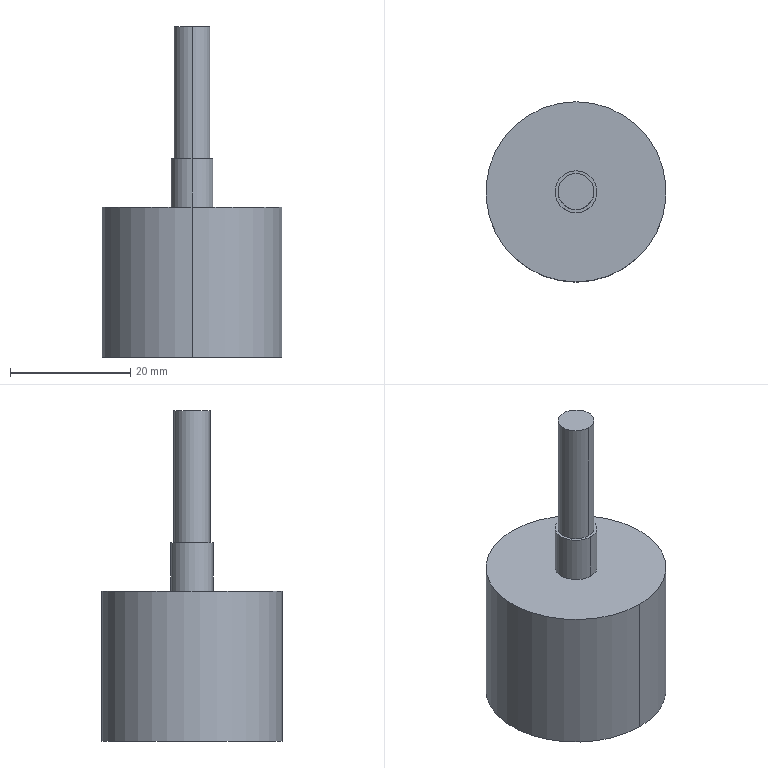Component | SolidWorks | LockingWheel-2 | 1 solid | 10 faces | box 30 x 30 x 55 mm | volume 18601 mm3 | cylinder 6 | plane 4 | commonest cylinder face diameters 6 x2 7 x2 30 x2
build123d program:
from build123d import *


with BuildPart() as part:
    # Sketch1 → Revolve1 (revolve)
    with BuildSketch(Plane.XY, mode=Mode.PRIVATE) as revolve1_sk:
        Polygon((0, 35.261), (15, 35.261), (15, 10.261), (3.5, 10.261), (3.5, 2.261), (3, 2.261), (3, -19.739), (0, -19.739), align=None)
    revolve(revolve1_sk.sketch.rotate(Axis((0, 0, 0), (0, 1, 0)), 90), axis=Axis((0, 0, 0), (0, 1, 0)))


solid = part.part

# Placed as in the assembly
solid = solid.moved(Location((-114.784, 711.983, -103.239), (-90, 0, 0)))
STEP:
#1=CARTESIAN_POINT('',(-4.519,27.913,-4.154));
#2=VERTEX_POINT('',#1);
#3=CARTESIAN_POINT('',(-4.519,28.149,-4.154));
#4=VERTEX_POINT('',#3);
#5=CARTESIAN_POINT('',(-4.519,28.031,-4.154));
#6=DIRECTION('',(0.,0.,1.));
#7=DIRECTION('',(0.,-1.,0.));
#8=AXIS2_PLACEMENT_3D('',#5,#6,#7);
#9=CIRCLE('',#8,0.1181);
#10=EDGE_CURVE('',#2,#4,#9,.T.);
#11=ORIENTED_EDGE('',*,*,#10,.T.);
#12=CARTESIAN_POINT('',(-4.519,28.149,-3.287));
#13=VERTEX_POINT('',#12);
#14=CARTESIAN_POINT('',(-4.519,28.149,-4.065));
#15=DIRECTION('',(0.,0.,1.));
#16=VECTOR('',#15,39.37);
#17=LINE('',#14,#16);
#18=EDGE_CURVE('',#4,#13,#17,.T.);
#19=ORIENTED_EDGE('',*,*,#18,.T.);
#20=CARTESIAN_POINT('',(-4.519,27.913,-3.287));
#21=VERTEX_POINT('',#20);
#22=CARTESIAN_POINT('',(-4.519,28.031,-3.287));
#23=DIRECTION('',(0.,0.,1.));
#24=DIRECTION('',(0.,-1.,0.));
#25=AXIS2_PLACEMENT_3D('',#22,#23,#24);
#26=CIRCLE('',#25,0.1181);
#27=EDGE_CURVE('',#21,#13,#26,.T.);
#28=ORIENTED_EDGE('',*,*,#27,.F.);
#29=CARTESIAN_POINT('',(-4.519,27.913,-4.065));
#30=DIRECTION('',(0.,0.,1.));
#31=VECTOR('',#30,39.37);
#32=LINE('',#29,#31);
#33=EDGE_CURVE('',#2,#21,#32,.T.);
#34=ORIENTED_EDGE('',*,*,#33,.F.);
#35=EDGE_LOOP('',(#11,#19,#28,#34));
#36=FACE_OUTER_BOUND('',#35,.T.);
#37=CARTESIAN_POINT('',(-4.519,28.031,-4.065));
#38=DIRECTION('',(0.,0.,1.));
#39=DIRECTION('',(0.,-1.,0.));
#40=AXIS2_PLACEMENT_3D('',#37,#38,#39);
#41=CYLINDRICAL_SURFACE('',#40,0.1181);
#42=ADVANCED_FACE('',(#36),#41,.T.);
#43=CARTESIAN_POINT('',(-4.519,27.893,-4.469));
#44=VERTEX_POINT('',#43);
#45=CARTESIAN_POINT('',(-4.519,28.169,-4.469));
#46=VERTEX_POINT('',#45);
#47=CARTESIAN_POINT('',(-4.519,28.031,-4.469));
#48=DIRECTION('',(0.,0.,1.));
#49=DIRECTION('',(0.,-1.,0.));
#50=AXIS2_PLACEMENT_3D('',#47,#48,#49);
#51=CIRCLE('',#50,0.1378);
#52=EDGE_CURVE('',#44,#46,#51,.T.);
#53=ORIENTED_EDGE('',*,*,#52,.T.);
#54=CARTESIAN_POINT('',(-4.519,28.169,-4.154));
#55=VERTEX_POINT('',#54);
#56=CARTESIAN_POINT('',(-4.519,28.169,-4.065));
#57=DIRECTION('',(0.,0.,1.));
#58=VECTOR('',#57,39.37);
#59=LINE('',#56,#58);
#60=EDGE_CURVE('',#46,#55,#59,.T.);
#61=ORIENTED_EDGE('',*,*,#60,.T.);
#62=CARTESIAN_POINT('',(-4.519,27.893,-4.154));
#63=VERTEX_POINT('',#62);
#64=CARTESIAN_POINT('',(-4.519,28.031,-4.154));
#65=DIRECTION('',(0.,0.,1.));
#66=DIRECTION('',(0.,-1.,0.));
#67=AXIS2_PLACEMENT_3D('',#64,#65,#66);
#68=CIRCLE('',#67,0.1378);
#69=EDGE_CURVE('',#63,#55,#68,.T.);
#70=ORIENTED_EDGE('',*,*,#69,.F.);
#71=CARTESIAN_POINT('',(-4.519,27.893,-4.065));
#72=DIRECTION('',(0.,0.,1.));
#73=VECTOR('',#72,39.37);
#74=LINE('',#71,#73);
#75=EDGE_CURVE('',#44,#63,#74,.T.);
#76=ORIENTED_EDGE('',*,*,#75,.F.);
#77=EDGE_LOOP('',(#53,#61,#70,#76));
#78=FACE_OUTER_BOUND('',#77,.T.);
#79=CARTESIAN_POINT('',(-4.519,28.031,-4.065));
#80=DIRECTION('',(0.,0.,1.));
#81=DIRECTION('',(0.,-1.,0.));
#82=AXIS2_PLACEMENT_3D('',#79,#80,#81);
#83=CYLINDRICAL_SURFACE('',#82,0.1378);
#84=ADVANCED_FACE('',(#78),#83,.T.);
#85=CARTESIAN_POINT('',(-4.519,27.44,-5.453));
#86=VERTEX_POINT('',#85);
#87=CARTESIAN_POINT('',(-4.519,28.621,-5.453));
#88=VERTEX_POINT('',#87);
#89=CARTESIAN_POINT('',(-4.519,28.031,-5.453));
#90=DIRECTION('',(0.,0.,1.));
#91=DIRECTION('',(0.,-1.,0.));
#92=AXIS2_PLACEMENT_3D('',#89,#90,#91);
#93=CIRCLE('',#92,0.5906);
#94=EDGE_CURVE('',#86,#88,#93,.T.);
#95=ORIENTED_EDGE('',*,*,#94,.T.);
#96=CARTESIAN_POINT('',(-4.519,28.621,-4.469));
#97=VERTEX_POINT('',#96);
#98=CARTESIAN_POINT('',(-4.519,28.621,-4.065));
#99=DIRECTION('',(0.,0.,1.));
#100=VECTOR('',#99,39.37);
#101=LINE('',#98,#100);
#102=EDGE_CURVE('',#88,#97,#101,.T.);
#103=ORIENTED_EDGE('',*,*,#102,.T.);
#104=CARTESIAN_POINT('',(-4.519,27.44,-4.469));
#105=VERTEX_POINT('',#104);
#106=CARTESIAN_POINT('',(-4.519,28.031,-4.469));
#107=DIRECTION('',(0.,0.,1.));
#108=DIRECTION('',(0.,-1.,0.));
#109=AXIS2_PLACEMENT_3D('',#106,#107,#108);
#110=CIRCLE('',#109,0.5906);
#111=EDGE_CURVE('',#105,#97,#110,.T.);
#112=ORIENTED_EDGE('',*,*,#111,.F.);
#113=CARTESIAN_POINT('',(-4.519,27.44,-4.065));
#114=DIRECTION('',(0.,0.,1.));
#115=VECTOR('',#114,39.37);
#116=LINE('',#113,#115);
#117=EDGE_CURVE('',#86,#105,#116,.T.);
#118=ORIENTED_EDGE('',*,*,#117,.F.);
#119=EDGE_LOOP('',(#95,#103,#112,#118));
#120=FACE_OUTER_BOUND('',#119,.T.);
#121=CARTESIAN_POINT('',(-4.519,28.031,-4.065));
#122=DIRECTION('',(0.,0.,1.));
#123=DIRECTION('',(0.,-1.,0.));
#124=AXIS2_PLACEMENT_3D('',#121,#122,#123);
#125=CYLINDRICAL_SURFACE('',#124,0.5906);
#126=ADVANCED_FACE('',(#120),#125,.T.);
#127=ORIENTED_EDGE('',*,*,#94,.F.);
#128=CARTESIAN_POINT('',(-4.519,28.031,-5.453));
#129=DIRECTION('',(0.,0.,1.));
#130=DIRECTION('',(0.,-1.,0.));
#131=AXIS2_PLACEMENT_3D('',#128,#129,#130);
#132=CIRCLE('',#131,0.5906);
#133=EDGE_CURVE('',#88,#86,#132,.T.);
#134=ORIENTED_EDGE('',*,*,#133,.F.);
#135=EDGE_LOOP('',(#127,#134));
#136=FACE_OUTER_BOUND('',#135,.T.);
#137=CARTESIAN_POINT('',(-4.519,28.031,-5.453));
#138=DIRECTION('',(-0.,-0.,-1.));
#139=DIRECTION('',(-0.,1.,-0.));
#140=AXIS2_PLACEMENT_3D('',#137,#138,#139);
#141=PLANE('',#140);
#142=ADVANCED_FACE('',(#136),#141,.T.);
#143=ORIENTED_EDGE('',*,*,#102,.F.);
#144=ORIENTED_EDGE('',*,*,#133,.T.);
#145=ORIENTED_EDGE('',*,*,#117,.T.);
#146=CARTESIAN_POINT('',(-4.519,28.031,-4.469));
#147=DIRECTION('',(0.,0.,1.));
#148=DIRECTION('',(0.,-1.,0.));
#149=AXIS2_PLACEMENT_3D('',#146,#147,#148);
#150=CIRCLE('',#149,0.5906);
#151=EDGE_CURVE('',#97,#105,#150,.T.);
#152=ORIENTED_EDGE('',*,*,#151,.F.);
#153=EDGE_LOOP('',(#143,#144,#145,#152));
#154=FACE_OUTER_BOUND('',#153,.T.);
#155=CARTESIAN_POINT('',(-4.519,28.031,-4.065));
#156=DIRECTION('',(0.,0.,1.));
#157=DIRECTION('',(0.,-1.,0.));
#158=AXIS2_PLACEMENT_3D('',#155,#156,#157);
#159=CYLINDRICAL_SURFACE('',#158,0.5906);
#160=ADVANCED_FACE('',(#154),#159,.T.);
#161=ORIENTED_EDGE('',*,*,#111,.T.);
#162=ORIENTED_EDGE('',*,*,#151,.T.);
#163=EDGE_LOOP('',(#161,#162));
#164=FACE_OUTER_BOUND('',#163,.T.);
#165=ORIENTED_EDGE('',*,*,#52,.F.);
#166=CARTESIAN_POINT('',(-4.519,28.031,-4.469));
#167=DIRECTION('',(0.,0.,1.));
#168=DIRECTION('',(0.,-1.,0.));
#169=AXIS2_PLACEMENT_3D('',#166,#167,#168);
#170=CIRCLE('',#169,0.1378);
#171=EDGE_CURVE('',#46,#44,#170,.T.);
#172=ORIENTED_EDGE('',*,*,#171,.F.);
#173=EDGE_LOOP('',(#165,#172));
#174=FACE_BOUND('',#173,.T.);
#175=CARTESIAN_POINT('',(-3.928,28.031,-4.469));
#176=DIRECTION('',(0.,0.,1.));
#177=DIRECTION('',(0.,-1.,0.));
#178=AXIS2_PLACEMENT_3D('',#175,#176,#177);
#179=PLANE('',#178);
#180=ADVANCED_FACE('',(#164,#174),#179,.T.);
#181=ORIENTED_EDGE('',*,*,#60,.F.);
#182=ORIENTED_EDGE('',*,*,#171,.T.);
#183=ORIENTED_EDGE('',*,*,#75,.T.);
#184=CARTESIAN_POINT('',(-4.519,28.031,-4.154));
#185=DIRECTION('',(0.,0.,1.));
#186=DIRECTION('',(0.,-1.,0.));
#187=AXIS2_PLACEMENT_3D('',#184,#185,#186);
#188=CIRCLE('',#187,0.1378);
#189=EDGE_CURVE('',#55,#63,#188,.T.);
#190=ORIENTED_EDGE('',*,*,#189,.F.);
#191=EDGE_LOOP('',(#181,#182,#183,#190));
#192=FACE_OUTER_BOUND('',#191,.T.);
#193=CARTESIAN_POINT('',(-4.519,28.031,-4.065));
#194=DIRECTION('',(0.,0.,1.));
#195=DIRECTION('',(0.,-1.,0.));
#196=AXIS2_PLACEMENT_3D('',#193,#194,#195);
#197=CYLINDRICAL_SURFACE('',#196,0.1378);
#198=ADVANCED_FACE('',(#192),#197,.T.);
#199=ORIENTED_EDGE('',*,*,#69,.T.);
#200=ORIENTED_EDGE('',*,*,#189,.T.);
#201=EDGE_LOOP('',(#199,#200));
#202=FACE_OUTER_BOUND('',#201,.T.);
#203=ORIENTED_EDGE('',*,*,#10,.F.);
#204=CARTESIAN_POINT('',(-4.519,28.031,-4.154));
#205=DIRECTION('',(0.,0.,1.));
#206=DIRECTION('',(0.,-1.,0.));
#207=AXIS2_PLACEMENT_3D('',#204,#205,#206);
#208=CIRCLE('',#207,0.1181);
#209=EDGE_CURVE('',#4,#2,#208,.T.);
#210=ORIENTED_EDGE('',*,*,#209,.F.);
#211=EDGE_LOOP('',(#203,#210));
#212=FACE_BOUND('',#211,.T.);
#213=CARTESIAN_POINT('',(-4.381,28.031,-4.154));
#214=DIRECTION('',(0.,0.,1.));
#215=DIRECTION('',(0.,-1.,0.));
#216=AXIS2_PLACEMENT_3D('',#213,#214,#215);
#217=PLANE('',#216);
#218=ADVANCED_FACE('',(#202,#212),#217,.T.);
#219=ORIENTED_EDGE('',*,*,#18,.F.);
#220=ORIENTED_EDGE('',*,*,#209,.T.);
#221=ORIENTED_EDGE('',*,*,#33,.T.);
#222=CARTESIAN_POINT('',(-4.519,28.031,-3.287));
#223=DIRECTION('',(0.,0.,1.));
#224=DIRECTION('',(0.,-1.,0.));
#225=AXIS2_PLACEMENT_3D('',#222,#223,#224);
#226=CIRCLE('',#225,0.1181);
#227=EDGE_CURVE('',#13,#21,#226,.T.);
#228=ORIENTED_EDGE('',*,*,#227,.F.);
#229=EDGE_LOOP('',(#219,#220,#221,#228));
#230=FACE_OUTER_BOUND('',#229,.T.);
#231=CARTESIAN_POINT('',(-4.519,28.031,-4.065));
#232=DIRECTION('',(0.,0.,1.));
#233=DIRECTION('',(0.,-1.,0.));
#234=AXIS2_PLACEMENT_3D('',#231,#232,#233);
#235=CYLINDRICAL_SURFACE('',#234,0.1181);
#236=ADVANCED_FACE('',(#230),#235,.T.);
#237=ORIENTED_EDGE('',*,*,#27,.T.);
#238=ORIENTED_EDGE('',*,*,#227,.T.);
#239=EDGE_LOOP('',(#237,#238));
#240=FACE_OUTER_BOUND('',#239,.T.);
#241=CARTESIAN_POINT('',(-4.401,28.031,-3.287));
#242=DIRECTION('',(0.,0.,1.));
#243=DIRECTION('',(0.,-1.,0.));
#244=AXIS2_PLACEMENT_3D('',#241,#242,#243);
#245=PLANE('',#244);
#246=ADVANCED_FACE('',(#240),#245,.T.);
#247=CLOSED_SHELL('',(#42,#84,#126,#142,#160,#180,#198,#218,#236,#246));
#248=MANIFOLD_SOLID_BREP('',#247);
#249=CARTESIAN_POINT('',(0.,0.,0.));
#250=DIRECTION('',(0.,0.,1.));
#251=DIRECTION('',(1.,0.,0.));
#252=AXIS2_PLACEMENT_3D('',#249,#250,#251);
#253=(LENGTH_UNIT()NAMED_UNIT(*)SI_UNIT($,.METRE.));
#254=LENGTH_MEASURE_WITH_UNIT(LENGTH_MEASURE(0.0254),#253);
#255=DIMENSIONAL_EXPONENTS(1.,0.,0.,0.,0.,0.,0.);
#256=(CONVERSION_BASED_UNIT('',#254)LENGTH_UNIT()NAMED_UNIT(#255));
#257=UNCERTAINTY_MEASURE_WITH_UNIT(LENGTH_MEASURE(0.00001),#256,'','');
#258=(NAMED_UNIT(*)PLANE_ANGLE_UNIT()SI_UNIT($,.RADIAN.));
#259=(NAMED_UNIT(*)SI_UNIT($,.STERADIAN.)SOLID_ANGLE_UNIT());
#260=(GEOMETRIC_REPRESENTATION_CONTEXT(3)GLOBAL_UNCERTAINTY_ASSIGNED_CONTEXT((#257))GLOBAL_UNIT_ASSIGNED_CONTEXT((#256,#258,#259))REPRESENTATION_CONTEXT('',''));
#261=ADVANCED_BREP_SHAPE_REPRESENTATION('',(#248,#252),#260);
#262=COLOUR_RGB('',0.7922,0.8196,0.9333);
#263=FILL_AREA_STYLE_COLOUR('',#262);
#264=FILL_AREA_STYLE('',(#263));
#265=SURFACE_STYLE_FILL_AREA(#264);
#266=SURFACE_SIDE_STYLE('',(#265));
#267=SURFACE_STYLE_USAGE(.BOTH.,#266);
#268=PRESENTATION_STYLE_ASSIGNMENT((#267));
#269=STYLED_ITEM('',(#268),#248);
#270=PRESENTATION_LAYER_ASSIGNMENT('','',(#269));
#271=(LENGTH_UNIT()NAMED_UNIT(*)SI_UNIT($,.METRE.));
#272=LENGTH_MEASURE_WITH_UNIT(LENGTH_MEASURE(0.0254),#271);
#273=DIMENSIONAL_EXPONENTS(1.,0.,0.,0.,0.,0.,0.);
#274=(CONVERSION_BASED_UNIT('',#272)LENGTH_UNIT()NAMED_UNIT(#273));
#275=UNCERTAINTY_MEASURE_WITH_UNIT(LENGTH_MEASURE(0.00001),#274,'','');
#276=(NAMED_UNIT(*)PLANE_ANGLE_UNIT()SI_UNIT($,.RADIAN.));
#277=(NAMED_UNIT(*)SI_UNIT($,.STERADIAN.)SOLID_ANGLE_UNIT());
#278=(GEOMETRIC_REPRESENTATION_CONTEXT(3)GLOBAL_UNCERTAINTY_ASSIGNED_CONTEXT((#275))GLOBAL_UNIT_ASSIGNED_CONTEXT((#274,#276,#277))REPRESENTATION_CONTEXT('',''));
#279=MECHANICAL_DESIGN_GEOMETRIC_PRESENTATION_REPRESENTATION('',(#269),#278);